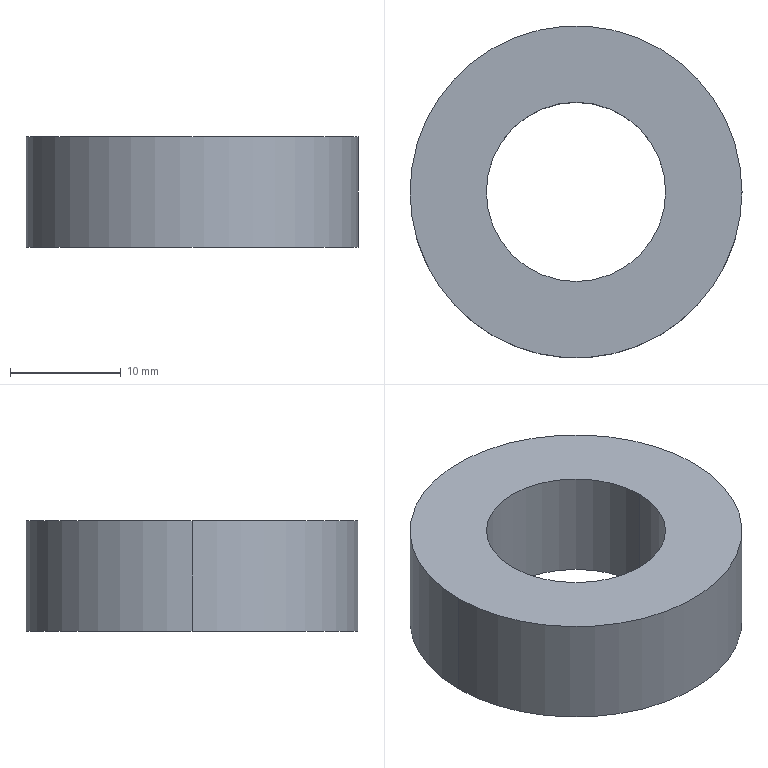Component | SolidWorks | YS01-058BufferPad-1 | 1 solid | 6 faces | box 30 x 30 x 10 mm | volume 5007 mm3 | cylinder 4 | plane 2 | commonest cylinder face diameters 16.2 x2 30 x2
build123d program:
from build123d import *

# Parameters (mm, degrees)
SKETCH1_R           = 15
SKETCH1_R_2         = 8.1
BOSS_EXTRUDE1_DEPTH = 10


with BuildPart() as part:
    # Sketch1 → Boss-Extrude1 (new body)
    with BuildSketch(Plane.XY):
        with Locations((-70, -20)):
            Circle(SKETCH1_R)
        with Locations((-70, -20)):
            Circle(SKETCH1_R_2, mode=Mode.SUBTRACT)
    extrude(amount=-BOSS_EXTRUDE1_DEPTH)


solid = part.part

# Placed as in the assembly
solid = solid.moved(Location((-426.612, -103.873, 2367.4), (0, 0, 0)))
STEP:
#1=COLOUR_RGB('',0.7922,0.8196,0.9333);
#2=FILL_AREA_STYLE_COLOUR('',#1);
#3=FILL_AREA_STYLE('',(#2));
#4=SURFACE_STYLE_FILL_AREA(#3);
#5=SURFACE_SIDE_STYLE('',(#4));
#6=SURFACE_STYLE_USAGE(.BOTH.,#5);
#7=PRESENTATION_STYLE_ASSIGNMENT((#6));
#8=CARTESIAN_POINT('',(-19.871,-4.877,93.205));
#9=VERTEX_POINT('',#8);
#10=CARTESIAN_POINT('',(-19.233,-4.877,93.205));
#11=VERTEX_POINT('',#10);
#12=CARTESIAN_POINT('',(-19.552,-4.877,93.205));
#13=DIRECTION('',(-0.,0.,-1.));
#14=DIRECTION('',(1.,0.,0.));
#15=AXIS2_PLACEMENT_3D('',#12,#13,#14);
#16=CIRCLE('',#15,0.3189);
#17=EDGE_CURVE('',#9,#11,#16,.T.);
#18=ORIENTED_EDGE('',*,*,#17,.F.);
#19=CARTESIAN_POINT('',(-19.871,-4.877,92.811));
#20=VERTEX_POINT('',#19);
#21=CARTESIAN_POINT('',(-19.871,-4.877,93.205));
#22=DIRECTION('',(-0.,0.,-1.));
#23=VECTOR('',#22,39.37);
#24=LINE('',#21,#23);
#25=EDGE_CURVE('',#9,#20,#24,.T.);
#26=ORIENTED_EDGE('',*,*,#25,.T.);
#27=CARTESIAN_POINT('',(-19.233,-4.877,92.811));
#28=VERTEX_POINT('',#27);
#29=CARTESIAN_POINT('',(-19.552,-4.877,92.811));
#30=DIRECTION('',(-0.,0.,-1.));
#31=DIRECTION('',(1.,0.,0.));
#32=AXIS2_PLACEMENT_3D('',#29,#30,#31);
#33=CIRCLE('',#32,0.3189);
#34=EDGE_CURVE('',#20,#28,#33,.T.);
#35=ORIENTED_EDGE('',*,*,#34,.T.);
#36=CARTESIAN_POINT('',(-19.233,-4.877,93.205));
#37=DIRECTION('',(-0.,0.,-1.));
#38=VECTOR('',#37,39.37);
#39=LINE('',#36,#38);
#40=EDGE_CURVE('',#11,#28,#39,.T.);
#41=ORIENTED_EDGE('',*,*,#40,.F.);
#42=EDGE_LOOP('',(#18,#26,#35,#41));
#43=FACE_OUTER_BOUND('',#42,.T.);
#44=CARTESIAN_POINT('',(-19.552,-4.877,93.205));
#45=DIRECTION('',(-0.,0.,-1.));
#46=DIRECTION('',(1.,0.,0.));
#47=AXIS2_PLACEMENT_3D('',#44,#45,#46);
#48=CYLINDRICAL_SURFACE('',#47,0.3189);
#49=ADVANCED_FACE('',(#43),#48,.F.);
#50=CARTESIAN_POINT('',(-18.961,-4.877,93.205));
#51=VERTEX_POINT('',#50);
#52=CARTESIAN_POINT('',(-20.142,-4.877,93.205));
#53=VERTEX_POINT('',#52);
#54=CARTESIAN_POINT('',(-19.552,-4.877,93.205));
#55=DIRECTION('',(-0.,0.,-1.));
#56=DIRECTION('',(1.,0.,0.));
#57=AXIS2_PLACEMENT_3D('',#54,#55,#56);
#58=CIRCLE('',#57,0.5906);
#59=EDGE_CURVE('',#51,#53,#58,.T.);
#60=ORIENTED_EDGE('',*,*,#59,.T.);
#61=CARTESIAN_POINT('',(-20.142,-4.877,92.811));
#62=VERTEX_POINT('',#61);
#63=CARTESIAN_POINT('',(-20.142,-4.877,93.205));
#64=DIRECTION('',(-0.,0.,-1.));
#65=VECTOR('',#64,39.37);
#66=LINE('',#63,#65);
#67=EDGE_CURVE('',#53,#62,#66,.T.);
#68=ORIENTED_EDGE('',*,*,#67,.T.);
#69=CARTESIAN_POINT('',(-18.961,-4.877,92.811));
#70=VERTEX_POINT('',#69);
#71=CARTESIAN_POINT('',(-19.552,-4.877,92.811));
#72=DIRECTION('',(-0.,0.,-1.));
#73=DIRECTION('',(1.,0.,0.));
#74=AXIS2_PLACEMENT_3D('',#71,#72,#73);
#75=CIRCLE('',#74,0.5906);
#76=EDGE_CURVE('',#70,#62,#75,.T.);
#77=ORIENTED_EDGE('',*,*,#76,.F.);
#78=CARTESIAN_POINT('',(-18.961,-4.877,93.205));
#79=DIRECTION('',(-0.,0.,-1.));
#80=VECTOR('',#79,39.37);
#81=LINE('',#78,#80);
#82=EDGE_CURVE('',#51,#70,#81,.T.);
#83=ORIENTED_EDGE('',*,*,#82,.F.);
#84=EDGE_LOOP('',(#60,#68,#77,#83));
#85=FACE_OUTER_BOUND('',#84,.T.);
#86=CARTESIAN_POINT('',(-19.552,-4.877,93.205));
#87=DIRECTION('',(-0.,0.,-1.));
#88=DIRECTION('',(1.,0.,0.));
#89=AXIS2_PLACEMENT_3D('',#86,#87,#88);
#90=CYLINDRICAL_SURFACE('',#89,0.5906);
#91=ADVANCED_FACE('',(#85),#90,.T.);
#92=ORIENTED_EDGE('',*,*,#67,.F.);
#93=CARTESIAN_POINT('',(-19.552,-4.877,93.205));
#94=DIRECTION('',(-0.,0.,-1.));
#95=DIRECTION('',(1.,0.,0.));
#96=AXIS2_PLACEMENT_3D('',#93,#94,#95);
#97=CIRCLE('',#96,0.5906);
#98=EDGE_CURVE('',#53,#51,#97,.T.);
#99=ORIENTED_EDGE('',*,*,#98,.T.);
#100=ORIENTED_EDGE('',*,*,#82,.T.);
#101=CARTESIAN_POINT('',(-19.552,-4.877,92.811));
#102=DIRECTION('',(-0.,0.,-1.));
#103=DIRECTION('',(1.,0.,0.));
#104=AXIS2_PLACEMENT_3D('',#101,#102,#103);
#105=CIRCLE('',#104,0.5906);
#106=EDGE_CURVE('',#62,#70,#105,.T.);
#107=ORIENTED_EDGE('',*,*,#106,.F.);
#108=EDGE_LOOP('',(#92,#99,#100,#107));
#109=FACE_OUTER_BOUND('',#108,.T.);
#110=CARTESIAN_POINT('',(-19.552,-4.877,93.205));
#111=DIRECTION('',(-0.,0.,-1.));
#112=DIRECTION('',(1.,0.,0.));
#113=AXIS2_PLACEMENT_3D('',#110,#111,#112);
#114=CYLINDRICAL_SURFACE('',#113,0.5906);
#115=ADVANCED_FACE('',(#109),#114,.T.);
#116=CARTESIAN_POINT('',(-19.552,-4.877,93.205));
#117=DIRECTION('',(-0.,0.,-1.));
#118=DIRECTION('',(1.,0.,0.));
#119=AXIS2_PLACEMENT_3D('',#116,#117,#118);
#120=CIRCLE('',#119,0.3189);
#121=EDGE_CURVE('',#11,#9,#120,.T.);
#122=ORIENTED_EDGE('',*,*,#121,.T.);
#123=ORIENTED_EDGE('',*,*,#17,.T.);
#124=EDGE_LOOP('',(#122,#123));
#125=FACE_BOUND('',#124,.T.);
#126=ORIENTED_EDGE('',*,*,#59,.F.);
#127=ORIENTED_EDGE('',*,*,#98,.F.);
#128=EDGE_LOOP('',(#126,#127));
#129=FACE_OUTER_BOUND('',#128,.T.);
#130=CARTESIAN_POINT('',(-19.552,-4.877,93.205));
#131=DIRECTION('',(-0.,0.,-1.));
#132=DIRECTION('',(1.,-0.,-0.));
#133=AXIS2_PLACEMENT_3D('',#130,#131,#132);
#134=PLANE('',#133);
#135=ADVANCED_FACE('',(#125,#129),#134,.F.);
#136=CARTESIAN_POINT('',(-19.552,-4.877,92.811));
#137=DIRECTION('',(-0.,0.,-1.));
#138=DIRECTION('',(1.,0.,0.));
#139=AXIS2_PLACEMENT_3D('',#136,#137,#138);
#140=CIRCLE('',#139,0.3189);
#141=EDGE_CURVE('',#28,#20,#140,.T.);
#142=ORIENTED_EDGE('',*,*,#141,.F.);
#143=ORIENTED_EDGE('',*,*,#34,.F.);
#144=EDGE_LOOP('',(#142,#143));
#145=FACE_BOUND('',#144,.T.);
#146=ORIENTED_EDGE('',*,*,#76,.T.);
#147=ORIENTED_EDGE('',*,*,#106,.T.);
#148=EDGE_LOOP('',(#146,#147));
#149=FACE_OUTER_BOUND('',#148,.T.);
#150=CARTESIAN_POINT('',(-19.552,-4.877,92.811));
#151=DIRECTION('',(-0.,0.,-1.));
#152=DIRECTION('',(1.,-0.,-0.));
#153=AXIS2_PLACEMENT_3D('',#150,#151,#152);
#154=PLANE('',#153);
#155=ADVANCED_FACE('',(#145,#149),#154,.T.);
#156=ORIENTED_EDGE('',*,*,#25,.F.);
#157=ORIENTED_EDGE('',*,*,#121,.F.);
#158=ORIENTED_EDGE('',*,*,#40,.T.);
#159=ORIENTED_EDGE('',*,*,#141,.T.);
#160=EDGE_LOOP('',(#156,#157,#158,#159));
#161=FACE_OUTER_BOUND('',#160,.T.);
#162=CARTESIAN_POINT('',(-19.552,-4.877,93.205));
#163=DIRECTION('',(-0.,0.,-1.));
#164=DIRECTION('',(1.,0.,0.));
#165=AXIS2_PLACEMENT_3D('',#162,#163,#164);
#166=CYLINDRICAL_SURFACE('',#165,0.3189);
#167=ADVANCED_FACE('',(#161),#166,.F.);
#168=CLOSED_SHELL('',(#49,#91,#115,#135,#155,#167));
#169=MANIFOLD_SOLID_BREP('',#168);
#170=STYLED_ITEM('',(#7),#169);
#171=PRESENTATION_LAYER_ASSIGNMENT('','',(#170));
#172=CARTESIAN_POINT('',(0.,0.,0.));
#173=DIRECTION('',(0.,0.,1.));
#174=DIRECTION('',(1.,0.,0.));
#175=AXIS2_PLACEMENT_3D('',#172,#173,#174);
#176=(LENGTH_UNIT()NAMED_UNIT(*)SI_UNIT($,.METRE.));
#177=LENGTH_MEASURE_WITH_UNIT(LENGTH_MEASURE(0.0254),#176);
#178=DIMENSIONAL_EXPONENTS(1.,0.,0.,0.,0.,0.,0.);
#179=(CONVERSION_BASED_UNIT('',#177)LENGTH_UNIT()NAMED_UNIT(#178));
#180=UNCERTAINTY_MEASURE_WITH_UNIT(LENGTH_MEASURE(0.00001),#179,'','');
#181=(NAMED_UNIT(*)PLANE_ANGLE_UNIT()SI_UNIT($,.RADIAN.));
#182=(NAMED_UNIT(*)SI_UNIT($,.STERADIAN.)SOLID_ANGLE_UNIT());
#183=(GEOMETRIC_REPRESENTATION_CONTEXT(3)GLOBAL_UNCERTAINTY_ASSIGNED_CONTEXT((#180))GLOBAL_UNIT_ASSIGNED_CONTEXT((#179,#181,#182))REPRESENTATION_CONTEXT('',''));
#184=ADVANCED_BREP_SHAPE_REPRESENTATION('',(#169,#175),#183);
#185=(LENGTH_UNIT()NAMED_UNIT(*)SI_UNIT($,.METRE.));
#186=LENGTH_MEASURE_WITH_UNIT(LENGTH_MEASURE(0.0254),#185);
#187=DIMENSIONAL_EXPONENTS(1.,0.,0.,0.,0.,0.,0.);
#188=(CONVERSION_BASED_UNIT('',#186)LENGTH_UNIT()NAMED_UNIT(#187));
#189=UNCERTAINTY_MEASURE_WITH_UNIT(LENGTH_MEASURE(0.00001),#188,'','');
#190=(NAMED_UNIT(*)PLANE_ANGLE_UNIT()SI_UNIT($,.RADIAN.));
#191=(NAMED_UNIT(*)SI_UNIT($,.STERADIAN.)SOLID_ANGLE_UNIT());
#192=(GEOMETRIC_REPRESENTATION_CONTEXT(3)GLOBAL_UNCERTAINTY_ASSIGNED_CONTEXT((#189))GLOBAL_UNIT_ASSIGNED_CONTEXT((#188,#190,#191))REPRESENTATION_CONTEXT('',''));
#193=MECHANICAL_DESIGN_GEOMETRIC_PRESENTATION_REPRESENTATION('',(#170),#192);